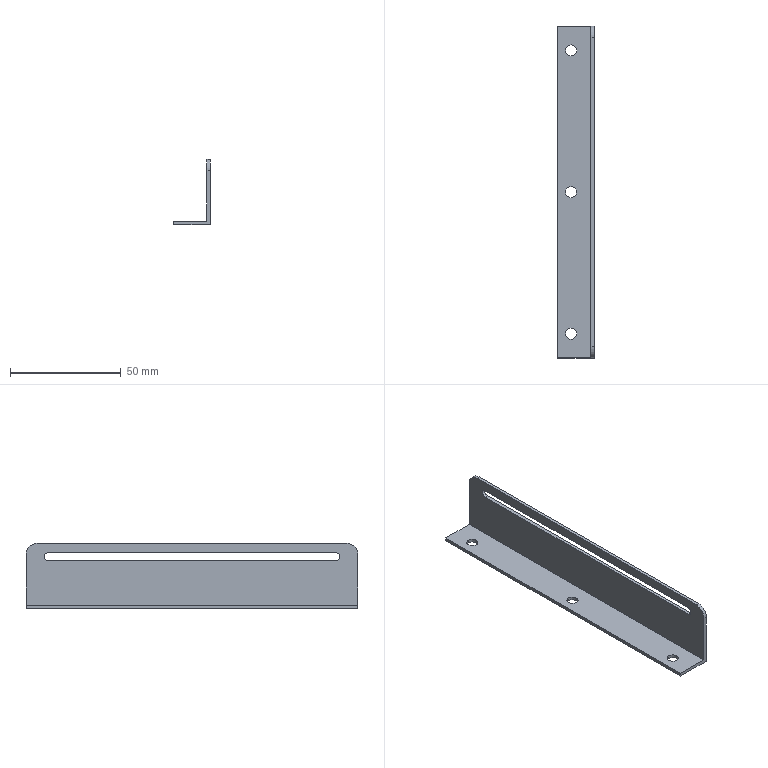Component | SolidWorks | DC-024-31-1 | 1 solid | 20 faces | box 16.5 x 150 x 29.5 mm | volume 9211 mm3 | cylinder 10 | plane 10 | commonest cylinder face diameters 5 x6 3.5 x2 10 x2
build123d program:
from build123d import *

# Parameters (mm, degrees)
EXTRUDE_THIN1_DEPTH      = 75
CUT_EXTRUDE1_DEPTH       = 10
F_5_0_5_DIAMETER_HOLE1_D = 5
FILLET1_R                = 5


with BuildPart() as part:
    # Sketch1 → Extrude-Thin1 (new, symmetric)
    with BuildSketch(Plane.XY):
        Polygon((0, 28), (0, 0), (-15, 0), (-15, -1.5), (1.5, -1.5), (1.5, 28), align=None)
    extrude(amount=EXTRUDE_THIN1_DEPTH, both=True)

    # Sketch2 → Cut-Extrude1 (cut)
    with BuildSketch(Plane.ZY):
        with BuildLine():
            Line((65, 20.25), (-65, 20.25))
            ThreePointArc((-65, 20.25), (-66.75, 22), (-65, 23.75))
            Line((-65, 23.75), (65, 23.75))
            ThreePointArc((65, 23.75), (66.75, 22), (65, 20.25))
        make_face()
    extrude(amount=-CUT_EXTRUDE1_DEPTH, mode=Mode.SUBTRACT)

    # 5.0 _5_ Diameter Hole1 (through all)
    with Locations(Plane(origin=(0, -1.5, 0), x_dir=(-1, 0, 0), z_dir=(0, -1, 0))):
        with Locations((9, 64), (9, 0), (9, -64)):
            Hole(F_5_0_5_DIAMETER_HOLE1_D / 2)

    # Fillet1
    fillet1_edges = [part.edges().sort_by_distance(p)[0] for p in [
        (0.75, 28, 75),
        (0.75, 28, -75),
    ]]
    fillet(fillet1_edges, radius=FILLET1_R)


solid = part.part

# Placed as in the assembly
solid = solid.moved(Location((112.867, 271.909, 14.5), (90, 0, 0)))
STEP:
#1=CARTESIAN_POINT('',(4.089,13.126,0.5709));
#2=VERTEX_POINT('',#1);
#3=CARTESIAN_POINT('',(4.089,13.323,0.5709));
#4=VERTEX_POINT('',#3);
#5=CARTESIAN_POINT('',(4.089,13.225,0.5709));
#6=DIRECTION('',(0.,0.,-1.));
#7=DIRECTION('',(1.,0.,0.));
#8=AXIS2_PLACEMENT_3D('',#5,#6,#7);
#9=CIRCLE('',#8,0.09843);
#10=EDGE_CURVE('',#2,#4,#9,.T.);
#11=ORIENTED_EDGE('',*,*,#10,.F.);
#12=CARTESIAN_POINT('',(4.089,13.126,0.5118));
#13=VERTEX_POINT('',#12);
#14=CARTESIAN_POINT('',(4.089,13.126,0.5118));
#15=DIRECTION('',(0.,0.,-1.));
#16=VECTOR('',#15,39.37);
#17=LINE('',#14,#16);
#18=EDGE_CURVE('',#2,#13,#17,.T.);
#19=ORIENTED_EDGE('',*,*,#18,.T.);
#20=CARTESIAN_POINT('',(4.089,13.323,0.5118));
#21=VERTEX_POINT('',#20);
#22=CARTESIAN_POINT('',(4.089,13.225,0.5118));
#23=DIRECTION('',(0.,0.,-1.));
#24=DIRECTION('',(0.,1.,0.));
#25=AXIS2_PLACEMENT_3D('',#22,#23,#24);
#26=CIRCLE('',#25,0.09843);
#27=EDGE_CURVE('',#13,#21,#26,.T.);
#28=ORIENTED_EDGE('',*,*,#27,.T.);
#29=CARTESIAN_POINT('',(4.089,13.323,0.5118));
#30=DIRECTION('',(0.,0.,-1.));
#31=VECTOR('',#30,39.37);
#32=LINE('',#29,#31);
#33=EDGE_CURVE('',#4,#21,#32,.T.);
#34=ORIENTED_EDGE('',*,*,#33,.F.);
#35=EDGE_LOOP('',(#11,#19,#28,#34));
#36=FACE_OUTER_BOUND('',#35,.T.);
#37=CARTESIAN_POINT('',(4.089,13.225,0.5118));
#38=DIRECTION('',(0.,0.,-1.));
#39=DIRECTION('',(0.,1.,0.));
#40=AXIS2_PLACEMENT_3D('',#37,#38,#39);
#41=CYLINDRICAL_SURFACE('',#40,0.09843);
#42=ADVANCED_FACE('',(#36),#41,.F.);
#43=CARTESIAN_POINT('',(4.089,10.607,0.5709));
#44=VERTEX_POINT('',#43);
#45=CARTESIAN_POINT('',(4.089,10.803,0.5709));
#46=VERTEX_POINT('',#45);
#47=CARTESIAN_POINT('',(4.089,10.705,0.5709));
#48=DIRECTION('',(0.,0.,-1.));
#49=DIRECTION('',(1.,0.,0.));
#50=AXIS2_PLACEMENT_3D('',#47,#48,#49);
#51=CIRCLE('',#50,0.09843);
#52=EDGE_CURVE('',#44,#46,#51,.T.);
#53=ORIENTED_EDGE('',*,*,#52,.F.);
#54=CARTESIAN_POINT('',(4.089,10.607,0.5118));
#55=VERTEX_POINT('',#54);
#56=CARTESIAN_POINT('',(4.089,10.607,0.5118));
#57=DIRECTION('',(0.,0.,-1.));
#58=VECTOR('',#57,39.37);
#59=LINE('',#56,#58);
#60=EDGE_CURVE('',#44,#55,#59,.T.);
#61=ORIENTED_EDGE('',*,*,#60,.T.);
#62=CARTESIAN_POINT('',(4.089,10.803,0.5118));
#63=VERTEX_POINT('',#62);
#64=CARTESIAN_POINT('',(4.089,10.705,0.5118));
#65=DIRECTION('',(0.,0.,-1.));
#66=DIRECTION('',(0.,1.,0.));
#67=AXIS2_PLACEMENT_3D('',#64,#65,#66);
#68=CIRCLE('',#67,0.09843);
#69=EDGE_CURVE('',#55,#63,#68,.T.);
#70=ORIENTED_EDGE('',*,*,#69,.T.);
#71=CARTESIAN_POINT('',(4.089,10.803,0.5118));
#72=DIRECTION('',(0.,0.,-1.));
#73=VECTOR('',#72,39.37);
#74=LINE('',#71,#73);
#75=EDGE_CURVE('',#46,#63,#74,.T.);
#76=ORIENTED_EDGE('',*,*,#75,.F.);
#77=EDGE_LOOP('',(#53,#61,#70,#76));
#78=FACE_OUTER_BOUND('',#77,.T.);
#79=CARTESIAN_POINT('',(4.089,10.705,0.5118));
#80=DIRECTION('',(0.,0.,-1.));
#81=DIRECTION('',(0.,1.,0.));
#82=AXIS2_PLACEMENT_3D('',#79,#80,#81);
#83=CYLINDRICAL_SURFACE('',#82,0.09843);
#84=ADVANCED_FACE('',(#78),#83,.F.);
#85=CARTESIAN_POINT('',(4.089,8.087,0.5709));
#86=VERTEX_POINT('',#85);
#87=CARTESIAN_POINT('',(4.089,8.284,0.5709));
#88=VERTEX_POINT('',#87);
#89=CARTESIAN_POINT('',(4.089,8.185,0.5709));
#90=DIRECTION('',(0.,0.,-1.));
#91=DIRECTION('',(1.,0.,0.));
#92=AXIS2_PLACEMENT_3D('',#89,#90,#91);
#93=CIRCLE('',#92,0.09843);
#94=EDGE_CURVE('',#86,#88,#93,.T.);
#95=ORIENTED_EDGE('',*,*,#94,.F.);
#96=CARTESIAN_POINT('',(4.089,8.087,0.5118));
#97=VERTEX_POINT('',#96);
#98=CARTESIAN_POINT('',(4.089,8.087,0.5118));
#99=DIRECTION('',(0.,0.,-1.));
#100=VECTOR('',#99,39.37);
#101=LINE('',#98,#100);
#102=EDGE_CURVE('',#86,#97,#101,.T.);
#103=ORIENTED_EDGE('',*,*,#102,.T.);
#104=CARTESIAN_POINT('',(4.089,8.284,0.5118));
#105=VERTEX_POINT('',#104);
#106=CARTESIAN_POINT('',(4.089,8.185,0.5118));
#107=DIRECTION('',(0.,0.,-1.));
#108=DIRECTION('',(0.,1.,0.));
#109=AXIS2_PLACEMENT_3D('',#106,#107,#108);
#110=CIRCLE('',#109,0.09843);
#111=EDGE_CURVE('',#97,#105,#110,.T.);
#112=ORIENTED_EDGE('',*,*,#111,.T.);
#113=CARTESIAN_POINT('',(4.089,8.284,0.5118));
#114=DIRECTION('',(0.,0.,-1.));
#115=VECTOR('',#114,39.37);
#116=LINE('',#113,#115);
#117=EDGE_CURVE('',#88,#105,#116,.T.);
#118=ORIENTED_EDGE('',*,*,#117,.F.);
#119=EDGE_LOOP('',(#95,#103,#112,#118));
#120=FACE_OUTER_BOUND('',#119,.T.);
#121=CARTESIAN_POINT('',(4.089,8.185,0.5118));
#122=DIRECTION('',(0.,0.,-1.));
#123=DIRECTION('',(0.,1.,0.));
#124=AXIS2_PLACEMENT_3D('',#121,#122,#123);
#125=CYLINDRICAL_SURFACE('',#124,0.09843);
#126=ADVANCED_FACE('',(#120),#125,.F.);
#127=CARTESIAN_POINT('',(4.089,13.225,0.5709));
#128=DIRECTION('',(0.,0.,-1.));
#129=DIRECTION('',(1.,0.,0.));
#130=AXIS2_PLACEMENT_3D('',#127,#128,#129);
#131=CIRCLE('',#130,0.09843);
#132=EDGE_CURVE('',#4,#2,#131,.T.);
#133=ORIENTED_EDGE('',*,*,#132,.T.);
#134=ORIENTED_EDGE('',*,*,#10,.T.);
#135=EDGE_LOOP('',(#133,#134));
#136=FACE_BOUND('',#135,.T.);
#137=CARTESIAN_POINT('',(4.089,10.705,0.5709));
#138=DIRECTION('',(0.,0.,-1.));
#139=DIRECTION('',(1.,0.,0.));
#140=AXIS2_PLACEMENT_3D('',#137,#138,#139);
#141=CIRCLE('',#140,0.09843);
#142=EDGE_CURVE('',#46,#44,#141,.T.);
#143=ORIENTED_EDGE('',*,*,#142,.T.);
#144=ORIENTED_EDGE('',*,*,#52,.T.);
#145=EDGE_LOOP('',(#143,#144));
#146=FACE_BOUND('',#145,.T.);
#147=CARTESIAN_POINT('',(4.089,8.185,0.5709));
#148=DIRECTION('',(0.,0.,-1.));
#149=DIRECTION('',(1.,0.,0.));
#150=AXIS2_PLACEMENT_3D('',#147,#148,#149);
#151=CIRCLE('',#150,0.09843);
#152=EDGE_CURVE('',#88,#86,#151,.T.);
#153=ORIENTED_EDGE('',*,*,#152,.T.);
#154=ORIENTED_EDGE('',*,*,#94,.T.);
#155=EDGE_LOOP('',(#153,#154));
#156=FACE_BOUND('',#155,.T.);
#157=CARTESIAN_POINT('',(4.444,13.658,0.5709));
#158=VERTEX_POINT('',#157);
#159=CARTESIAN_POINT('',(3.853,13.658,0.5709));
#160=VERTEX_POINT('',#159);
#161=CARTESIAN_POINT('',(4.444,13.658,0.5709));
#162=DIRECTION('',(-1.,0.,-0.));
#163=VECTOR('',#162,39.37);
#164=LINE('',#161,#163);
#165=EDGE_CURVE('',#158,#160,#164,.T.);
#166=ORIENTED_EDGE('',*,*,#165,.T.);
#167=CARTESIAN_POINT('',(3.853,7.752,0.5709));
#168=VERTEX_POINT('',#167);
#169=CARTESIAN_POINT('',(3.853,7.752,0.5709));
#170=DIRECTION('',(0.,1.,0.));
#171=VECTOR('',#170,39.37);
#172=LINE('',#169,#171);
#173=EDGE_CURVE('',#168,#160,#172,.T.);
#174=ORIENTED_EDGE('',*,*,#173,.F.);
#175=CARTESIAN_POINT('',(4.444,7.752,0.5709));
#176=VERTEX_POINT('',#175);
#177=CARTESIAN_POINT('',(4.444,7.752,0.5709));
#178=DIRECTION('',(-1.,0.,-0.));
#179=VECTOR('',#178,39.37);
#180=LINE('',#177,#179);
#181=EDGE_CURVE('',#176,#168,#180,.T.);
#182=ORIENTED_EDGE('',*,*,#181,.F.);
#183=CARTESIAN_POINT('',(4.444,7.752,0.5709));
#184=DIRECTION('',(0.,1.,0.));
#185=VECTOR('',#184,39.37);
#186=LINE('',#183,#185);
#187=EDGE_CURVE('',#176,#158,#186,.T.);
#188=ORIENTED_EDGE('',*,*,#187,.T.);
#189=EDGE_LOOP('',(#166,#174,#182,#188));
#190=FACE_OUTER_BOUND('',#189,.T.);
#191=CARTESIAN_POINT('',(4.444,7.752,0.5709));
#192=DIRECTION('',(0.,0.,-1.));
#193=DIRECTION('',(1.,0.,0.));
#194=AXIS2_PLACEMENT_3D('',#191,#192,#193);
#195=PLANE('',#194);
#196=ADVANCED_FACE('',(#136,#146,#156,#190),#195,.F.);
#197=CARTESIAN_POINT('',(3.853,13.658,0.5118));
#198=VERTEX_POINT('',#197);
#199=CARTESIAN_POINT('',(3.853,13.658,0.5118));
#200=DIRECTION('',(0.,0.,1.));
#201=VECTOR('',#200,39.37);
#202=LINE('',#199,#201);
#203=EDGE_CURVE('',#198,#160,#202,.T.);
#204=ORIENTED_EDGE('',*,*,#203,.F.);
#205=CARTESIAN_POINT('',(3.853,7.752,0.5118));
#206=VERTEX_POINT('',#205);
#207=CARTESIAN_POINT('',(3.853,7.752,0.5118));
#208=DIRECTION('',(0.,1.,0.));
#209=VECTOR('',#208,39.37);
#210=LINE('',#207,#209);
#211=EDGE_CURVE('',#206,#198,#210,.T.);
#212=ORIENTED_EDGE('',*,*,#211,.F.);
#213=CARTESIAN_POINT('',(3.853,7.752,0.5118));
#214=DIRECTION('',(0.,0.,1.));
#215=VECTOR('',#214,39.37);
#216=LINE('',#213,#215);
#217=EDGE_CURVE('',#206,#168,#216,.T.);
#218=ORIENTED_EDGE('',*,*,#217,.T.);
#219=ORIENTED_EDGE('',*,*,#173,.T.);
#220=EDGE_LOOP('',(#204,#212,#218,#219));
#221=FACE_OUTER_BOUND('',#220,.T.);
#222=CARTESIAN_POINT('',(3.853,7.752,0.5118));
#223=DIRECTION('',(-1.,0.,0.));
#224=DIRECTION('',(0.,-1.,0.));
#225=AXIS2_PLACEMENT_3D('',#222,#223,#224);
#226=PLANE('',#225);
#227=ADVANCED_FACE('',(#221),#226,.T.);
#228=CARTESIAN_POINT('',(4.089,13.225,0.5118));
#229=DIRECTION('',(0.,0.,-1.));
#230=DIRECTION('',(0.,1.,0.));
#231=AXIS2_PLACEMENT_3D('',#228,#229,#230);
#232=CIRCLE('',#231,0.09843);
#233=EDGE_CURVE('',#21,#13,#232,.T.);
#234=ORIENTED_EDGE('',*,*,#233,.F.);
#235=ORIENTED_EDGE('',*,*,#27,.F.);
#236=EDGE_LOOP('',(#234,#235));
#237=FACE_BOUND('',#236,.T.);
#238=CARTESIAN_POINT('',(4.089,10.705,0.5118));
#239=DIRECTION('',(0.,0.,-1.));
#240=DIRECTION('',(0.,1.,0.));
#241=AXIS2_PLACEMENT_3D('',#238,#239,#240);
#242=CIRCLE('',#241,0.09843);
#243=EDGE_CURVE('',#63,#55,#242,.T.);
#244=ORIENTED_EDGE('',*,*,#243,.F.);
#245=ORIENTED_EDGE('',*,*,#69,.F.);
#246=EDGE_LOOP('',(#244,#245));
#247=FACE_BOUND('',#246,.T.);
#248=CARTESIAN_POINT('',(4.089,8.185,0.5118));
#249=DIRECTION('',(0.,0.,-1.));
#250=DIRECTION('',(0.,1.,0.));
#251=AXIS2_PLACEMENT_3D('',#248,#249,#250);
#252=CIRCLE('',#251,0.09843);
#253=EDGE_CURVE('',#105,#97,#252,.T.);
#254=ORIENTED_EDGE('',*,*,#253,.F.);
#255=ORIENTED_EDGE('',*,*,#111,.F.);
#256=EDGE_LOOP('',(#254,#255));
#257=FACE_BOUND('',#256,.T.);
#258=CARTESIAN_POINT('',(4.503,13.658,0.5118));
#259=VERTEX_POINT('',#258);
#260=CARTESIAN_POINT('',(4.444,13.658,0.5118));
#261=DIRECTION('',(-1.,0.,-0.));
#262=VECTOR('',#261,39.37);
#263=LINE('',#260,#262);
#264=EDGE_CURVE('',#259,#198,#263,.T.);
#265=ORIENTED_EDGE('',*,*,#264,.F.);
#266=CARTESIAN_POINT('',(4.503,7.752,0.5118));
#267=VERTEX_POINT('',#266);
#268=CARTESIAN_POINT('',(4.503,7.752,0.5118));
#269=DIRECTION('',(0.,1.,0.));
#270=VECTOR('',#269,39.37);
#271=LINE('',#268,#270);
#272=EDGE_CURVE('',#267,#259,#271,.T.);
#273=ORIENTED_EDGE('',*,*,#272,.F.);
#274=CARTESIAN_POINT('',(4.444,7.752,0.5118));
#275=DIRECTION('',(-1.,0.,-0.));
#276=VECTOR('',#275,39.37);
#277=LINE('',#274,#276);
#278=EDGE_CURVE('',#267,#206,#277,.T.);
#279=ORIENTED_EDGE('',*,*,#278,.T.);
#280=ORIENTED_EDGE('',*,*,#211,.T.);
#281=EDGE_LOOP('',(#265,#273,#279,#280));
#282=FACE_OUTER_BOUND('',#281,.T.);
#283=CARTESIAN_POINT('',(4.444,7.752,0.5118));
#284=DIRECTION('',(0.,0.,-1.));
#285=DIRECTION('',(1.,0.,0.));
#286=AXIS2_PLACEMENT_3D('',#283,#284,#285);
#287=PLANE('',#286);
#288=ADVANCED_FACE('',(#237,#247,#257,#282),#287,.T.);
#289=CARTESIAN_POINT('',(4.503,8.146,1.506));
#290=VERTEX_POINT('',#289);
#291=CARTESIAN_POINT('',(4.503,8.146,1.368));
#292=VERTEX_POINT('',#291);
#293=CARTESIAN_POINT('',(4.503,8.146,1.437));
#294=DIRECTION('',(1.,0.,0.));
#295=DIRECTION('',(0.,0.,1.));
#296=AXIS2_PLACEMENT_3D('',#293,#294,#295);
#297=CIRCLE('',#296,0.0689);
#298=EDGE_CURVE('',#290,#292,#297,.T.);
#299=ORIENTED_EDGE('',*,*,#298,.F.);
#300=CARTESIAN_POINT('',(4.503,13.264,1.506));
#301=VERTEX_POINT('',#300);
#302=CARTESIAN_POINT('',(4.503,7.752,1.506));
#303=DIRECTION('',(0.,-1.,0.));
#304=VECTOR('',#303,39.37);
#305=LINE('',#302,#304);
#306=EDGE_CURVE('',#301,#290,#305,.T.);
#307=ORIENTED_EDGE('',*,*,#306,.F.);
#308=CARTESIAN_POINT('',(4.503,13.264,1.368));
#309=VERTEX_POINT('',#308);
#310=CARTESIAN_POINT('',(4.503,13.264,1.437));
#311=DIRECTION('',(1.,0.,0.));
#312=DIRECTION('',(0.,0.,1.));
#313=AXIS2_PLACEMENT_3D('',#310,#311,#312);
#314=CIRCLE('',#313,0.0689);
#315=EDGE_CURVE('',#309,#301,#314,.T.);
#316=ORIENTED_EDGE('',*,*,#315,.F.);
#317=CARTESIAN_POINT('',(4.503,7.752,1.368));
#318=DIRECTION('',(0.,1.,-0.));
#319=VECTOR('',#318,39.37);
#320=LINE('',#317,#319);
#321=EDGE_CURVE('',#292,#309,#320,.T.);
#322=ORIENTED_EDGE('',*,*,#321,.F.);
#323=EDGE_LOOP('',(#299,#307,#316,#322));
#324=FACE_BOUND('',#323,.T.);
#325=CARTESIAN_POINT('',(4.503,13.658,1.476));
#326=VERTEX_POINT('',#325);
#327=CARTESIAN_POINT('',(4.503,13.658,1.673));
#328=DIRECTION('',(0.,0.,-1.));
#329=VECTOR('',#328,39.37);
#330=LINE('',#327,#329);
#331=EDGE_CURVE('',#326,#259,#330,.T.);
#332=ORIENTED_EDGE('',*,*,#331,.F.);
#333=CARTESIAN_POINT('',(4.503,13.461,1.673));
#334=VERTEX_POINT('',#333);
#335=CARTESIAN_POINT('',(4.503,13.461,1.476));
#336=DIRECTION('',(1.,0.,0.));
#337=DIRECTION('',(0.,0.,1.));
#338=AXIS2_PLACEMENT_3D('',#335,#336,#337);
#339=CIRCLE('',#338,0.1969);
#340=EDGE_CURVE('',#326,#334,#339,.T.);
#341=ORIENTED_EDGE('',*,*,#340,.T.);
#342=CARTESIAN_POINT('',(4.503,7.949,1.673));
#343=VERTEX_POINT('',#342);
#344=CARTESIAN_POINT('',(4.503,7.752,1.673));
#345=DIRECTION('',(0.,1.,0.));
#346=VECTOR('',#345,39.37);
#347=LINE('',#344,#346);
#348=EDGE_CURVE('',#343,#334,#347,.T.);
#349=ORIENTED_EDGE('',*,*,#348,.F.);
#350=CARTESIAN_POINT('',(4.503,7.752,1.476));
#351=VERTEX_POINT('',#350);
#352=CARTESIAN_POINT('',(4.503,7.949,1.476));
#353=DIRECTION('',(1.,0.,0.));
#354=DIRECTION('',(0.,0.,1.));
#355=AXIS2_PLACEMENT_3D('',#352,#353,#354);
#356=CIRCLE('',#355,0.1969);
#357=EDGE_CURVE('',#343,#351,#356,.T.);
#358=ORIENTED_EDGE('',*,*,#357,.T.);
#359=CARTESIAN_POINT('',(4.503,7.752,1.673));
#360=DIRECTION('',(0.,0.,-1.));
#361=VECTOR('',#360,39.37);
#362=LINE('',#359,#361);
#363=EDGE_CURVE('',#351,#267,#362,.T.);
#364=ORIENTED_EDGE('',*,*,#363,.T.);
#365=ORIENTED_EDGE('',*,*,#272,.T.);
#366=EDGE_LOOP('',(#332,#341,#349,#358,#364,#365));
#367=FACE_OUTER_BOUND('',#366,.T.);
#368=CARTESIAN_POINT('',(4.503,7.752,1.673));
#369=DIRECTION('',(1.,0.,0.));
#370=DIRECTION('',(-0.,0.,1.));
#371=AXIS2_PLACEMENT_3D('',#368,#369,#370);
#372=PLANE('',#371);
#373=ADVANCED_FACE('',(#324,#367),#372,.T.);
#374=ORIENTED_EDGE('',*,*,#348,.T.);
#375=CARTESIAN_POINT('',(4.444,13.461,1.673));
#376=VERTEX_POINT('',#375);
#377=CARTESIAN_POINT('',(4.444,13.461,1.673));
#378=DIRECTION('',(-1.,0.,0.));
#379=VECTOR('',#378,39.37);
#380=LINE('',#377,#379);
#381=EDGE_CURVE('',#334,#376,#380,.T.);
#382=ORIENTED_EDGE('',*,*,#381,.T.);
#383=CARTESIAN_POINT('',(4.444,7.949,1.673));
#384=VERTEX_POINT('',#383);
#385=CARTESIAN_POINT('',(4.444,7.752,1.673));
#386=DIRECTION('',(0.,1.,0.));
#387=VECTOR('',#386,39.37);
#388=LINE('',#385,#387);
#389=EDGE_CURVE('',#384,#376,#388,.T.);
#390=ORIENTED_EDGE('',*,*,#389,.F.);
#391=CARTESIAN_POINT('',(4.503,7.949,1.673));
#392=DIRECTION('',(1.,0.,0.));
#393=VECTOR('',#392,39.37);
#394=LINE('',#391,#393);
#395=EDGE_CURVE('',#384,#343,#394,.T.);
#396=ORIENTED_EDGE('',*,*,#395,.T.);
#397=EDGE_LOOP('',(#374,#382,#390,#396));
#398=FACE_OUTER_BOUND('',#397,.T.);
#399=CARTESIAN_POINT('',(4.444,7.752,1.673));
#400=DIRECTION('',(0.,0.,1.));
#401=DIRECTION('',(0.,-1.,0.));
#402=AXIS2_PLACEMENT_3D('',#399,#400,#401);
#403=PLANE('',#402);
#404=ADVANCED_FACE('',(#398),#403,.T.);
#405=CARTESIAN_POINT('',(4.444,8.146,1.506));
#406=VERTEX_POINT('',#405);
#407=CARTESIAN_POINT('',(4.444,13.264,1.506));
#408=VERTEX_POINT('',#407);
#409=CARTESIAN_POINT('',(4.444,8.146,1.506));
#410=DIRECTION('',(0.,1.,0.));
#411=VECTOR('',#410,39.37);
#412=LINE('',#409,#411);
#413=EDGE_CURVE('',#406,#408,#412,.T.);
#414=ORIENTED_EDGE('',*,*,#413,.F.);
#415=CARTESIAN_POINT('',(4.444,8.146,1.368));
#416=VERTEX_POINT('',#415);
#417=CARTESIAN_POINT('',(4.444,8.146,1.437));
#418=DIRECTION('',(-1.,0.,0.));
#419=DIRECTION('',(0.,0.,-1.));
#420=AXIS2_PLACEMENT_3D('',#417,#418,#419);
#421=CIRCLE('',#420,0.0689);
#422=EDGE_CURVE('',#416,#406,#421,.T.);
#423=ORIENTED_EDGE('',*,*,#422,.F.);
#424=CARTESIAN_POINT('',(4.444,13.264,1.368));
#425=VERTEX_POINT('',#424);
#426=CARTESIAN_POINT('',(4.444,8.146,1.368));
#427=DIRECTION('',(0.,-1.,0.));
#428=VECTOR('',#427,39.37);
#429=LINE('',#426,#428);
#430=EDGE_CURVE('',#425,#416,#429,.T.);
#431=ORIENTED_EDGE('',*,*,#430,.F.);
#432=CARTESIAN_POINT('',(4.444,13.264,1.437));
#433=DIRECTION('',(-1.,0.,0.));
#434=DIRECTION('',(0.,0.,-1.));
#435=AXIS2_PLACEMENT_3D('',#432,#433,#434);
#436=CIRCLE('',#435,0.0689);
#437=EDGE_CURVE('',#408,#425,#436,.T.);
#438=ORIENTED_EDGE('',*,*,#437,.F.);
#439=EDGE_LOOP('',(#414,#423,#431,#438));
#440=FACE_BOUND('',#439,.T.);
#441=ORIENTED_EDGE('',*,*,#389,.T.);
#442=CARTESIAN_POINT('',(4.444,13.658,1.476));
#443=VERTEX_POINT('',#442);
#444=CARTESIAN_POINT('',(4.444,13.461,1.476));
#445=DIRECTION('',(-1.,0.,-0.));
#446=DIRECTION('',(0.,0.,1.));
#447=AXIS2_PLACEMENT_3D('',#444,#445,#446);
#448=CIRCLE('',#447,0.1969);
#449=EDGE_CURVE('',#376,#443,#448,.T.);
#450=ORIENTED_EDGE('',*,*,#449,.T.);
#451=CARTESIAN_POINT('',(4.444,13.658,1.673));
#452=DIRECTION('',(0.,0.,-1.));
#453=VECTOR('',#452,39.37);
#454=LINE('',#451,#453);
#455=EDGE_CURVE('',#443,#158,#454,.T.);
#456=ORIENTED_EDGE('',*,*,#455,.T.);
#457=ORIENTED_EDGE('',*,*,#187,.F.);
#458=CARTESIAN_POINT('',(4.444,7.752,1.476));
#459=VERTEX_POINT('',#458);
#460=CARTESIAN_POINT('',(4.444,7.752,1.673));
#461=DIRECTION('',(0.,0.,-1.));
#462=VECTOR('',#461,39.37);
#463=LINE('',#460,#462);
#464=EDGE_CURVE('',#459,#176,#463,.T.);
#465=ORIENTED_EDGE('',*,*,#464,.F.);
#466=CARTESIAN_POINT('',(4.444,7.949,1.476));
#467=DIRECTION('',(-1.,0.,-0.));
#468=DIRECTION('',(0.,0.,1.));
#469=AXIS2_PLACEMENT_3D('',#466,#467,#468);
#470=CIRCLE('',#469,0.1969);
#471=EDGE_CURVE('',#459,#384,#470,.T.);
#472=ORIENTED_EDGE('',*,*,#471,.T.);
#473=EDGE_LOOP('',(#441,#450,#456,#457,#465,#472));
#474=FACE_OUTER_BOUND('',#473,.T.);
#475=CARTESIAN_POINT('',(4.444,7.752,1.673));
#476=DIRECTION('',(1.,0.,0.));
#477=DIRECTION('',(-0.,0.,1.));
#478=AXIS2_PLACEMENT_3D('',#475,#476,#477);
#479=PLANE('',#478);
#480=ADVANCED_FACE('',(#440,#474),#479,.F.);
#481=ORIENTED_EDGE('',*,*,#363,.F.);
#482=CARTESIAN_POINT('',(4.444,7.752,1.476));
#483=DIRECTION('',(-1.,0.,0.));
#484=VECTOR('',#483,39.37);
#485=LINE('',#482,#484);
#486=EDGE_CURVE('',#351,#459,#485,.T.);
#487=ORIENTED_EDGE('',*,*,#486,.T.);
#488=ORIENTED_EDGE('',*,*,#464,.T.);
#489=ORIENTED_EDGE('',*,*,#181,.T.);
#490=ORIENTED_EDGE('',*,*,#217,.F.);
#491=ORIENTED_EDGE('',*,*,#278,.F.);
#492=EDGE_LOOP('',(#481,#487,#488,#489,#490,#491));
#493=FACE_OUTER_BOUND('',#492,.T.);
#494=CARTESIAN_POINT('',(4.444,7.752,0.5709));
#495=DIRECTION('',(0.,1.,0.));
#496=DIRECTION('',(-1.,0.,0.));
#497=AXIS2_PLACEMENT_3D('',#494,#495,#496);
#498=PLANE('',#497);
#499=ADVANCED_FACE('',(#493),#498,.F.);
#500=ORIENTED_EDGE('',*,*,#455,.F.);
#501=CARTESIAN_POINT('',(4.444,13.658,1.476));
#502=DIRECTION('',(1.,0.,0.));
#503=VECTOR('',#502,39.37);
#504=LINE('',#501,#503);
#505=EDGE_CURVE('',#443,#326,#504,.T.);
#506=ORIENTED_EDGE('',*,*,#505,.T.);
#507=ORIENTED_EDGE('',*,*,#331,.T.);
#508=ORIENTED_EDGE('',*,*,#264,.T.);
#509=ORIENTED_EDGE('',*,*,#203,.T.);
#510=ORIENTED_EDGE('',*,*,#165,.F.);
#511=EDGE_LOOP('',(#500,#506,#507,#508,#509,#510));
#512=FACE_OUTER_BOUND('',#511,.T.);
#513=CARTESIAN_POINT('',(4.444,13.658,0.5709));
#514=DIRECTION('',(0.,1.,0.));
#515=DIRECTION('',(-1.,0.,0.));
#516=AXIS2_PLACEMENT_3D('',#513,#514,#515);
#517=PLANE('',#516);
#518=ADVANCED_FACE('',(#512),#517,.T.);
#519=ORIENTED_EDGE('',*,*,#298,.T.);
#520=CARTESIAN_POINT('',(4.837,8.146,1.368));
#521=DIRECTION('',(-1.,0.,0.));
#522=VECTOR('',#521,39.37);
#523=LINE('',#520,#522);
#524=EDGE_CURVE('',#292,#416,#523,.T.);
#525=ORIENTED_EDGE('',*,*,#524,.T.);
#526=ORIENTED_EDGE('',*,*,#422,.T.);
#527=CARTESIAN_POINT('',(4.837,8.146,1.506));
#528=DIRECTION('',(-1.,0.,0.));
#529=VECTOR('',#528,39.37);
#530=LINE('',#527,#529);
#531=EDGE_CURVE('',#290,#406,#530,.T.);
#532=ORIENTED_EDGE('',*,*,#531,.F.);
#533=EDGE_LOOP('',(#519,#525,#526,#532));
#534=FACE_OUTER_BOUND('',#533,.T.);
#535=CARTESIAN_POINT('',(4.837,8.146,1.437));
#536=DIRECTION('',(-1.,0.,0.));
#537=DIRECTION('',(0.,0.,-1.));
#538=AXIS2_PLACEMENT_3D('',#535,#536,#537);
#539=CYLINDRICAL_SURFACE('',#538,0.0689);
#540=ADVANCED_FACE('',(#534),#539,.F.);
#541=ORIENTED_EDGE('',*,*,#321,.T.);
#542=CARTESIAN_POINT('',(4.837,13.264,1.368));
#543=DIRECTION('',(-1.,0.,0.));
#544=VECTOR('',#543,39.37);
#545=LINE('',#542,#544);
#546=EDGE_CURVE('',#309,#425,#545,.T.);
#547=ORIENTED_EDGE('',*,*,#546,.T.);
#548=ORIENTED_EDGE('',*,*,#430,.T.);
#549=ORIENTED_EDGE('',*,*,#524,.F.);
#550=EDGE_LOOP('',(#541,#547,#548,#549));
#551=FACE_OUTER_BOUND('',#550,.T.);
#552=CARTESIAN_POINT('',(4.837,8.146,1.368));
#553=DIRECTION('',(-0.,-0.,-1.));
#554=DIRECTION('',(0.,1.,-0.));
#555=AXIS2_PLACEMENT_3D('',#552,#553,#554);
#556=PLANE('',#555);
#557=ADVANCED_FACE('',(#551),#556,.F.);
#558=ORIENTED_EDGE('',*,*,#315,.T.);
#559=CARTESIAN_POINT('',(4.837,13.264,1.506));
#560=DIRECTION('',(-1.,0.,0.));
#561=VECTOR('',#560,39.37);
#562=LINE('',#559,#561);
#563=EDGE_CURVE('',#301,#408,#562,.T.);
#564=ORIENTED_EDGE('',*,*,#563,.T.);
#565=ORIENTED_EDGE('',*,*,#437,.T.);
#566=ORIENTED_EDGE('',*,*,#546,.F.);
#567=EDGE_LOOP('',(#558,#564,#565,#566));
#568=FACE_OUTER_BOUND('',#567,.T.);
#569=CARTESIAN_POINT('',(4.837,13.264,1.437));
#570=DIRECTION('',(-1.,0.,0.));
#571=DIRECTION('',(0.,0.,-1.));
#572=AXIS2_PLACEMENT_3D('',#569,#570,#571);
#573=CYLINDRICAL_SURFACE('',#572,0.0689);
#574=ADVANCED_FACE('',(#568),#573,.F.);
#575=ORIENTED_EDGE('',*,*,#306,.T.);
#576=ORIENTED_EDGE('',*,*,#531,.T.);
#577=ORIENTED_EDGE('',*,*,#413,.T.);
#578=ORIENTED_EDGE('',*,*,#563,.F.);
#579=EDGE_LOOP('',(#575,#576,#577,#578));
#580=FACE_OUTER_BOUND('',#579,.T.);
#581=CARTESIAN_POINT('',(4.837,8.146,1.506));
#582=DIRECTION('',(0.,0.,1.));
#583=DIRECTION('',(-1.,0.,0.));
#584=AXIS2_PLACEMENT_3D('',#581,#582,#583);
#585=PLANE('',#584);
#586=ADVANCED_FACE('',(#580),#585,.F.);
#587=ORIENTED_EDGE('',*,*,#102,.F.);
#588=ORIENTED_EDGE('',*,*,#152,.F.);
#589=ORIENTED_EDGE('',*,*,#117,.T.);
#590=ORIENTED_EDGE('',*,*,#253,.T.);
#591=EDGE_LOOP('',(#587,#588,#589,#590));
#592=FACE_OUTER_BOUND('',#591,.T.);
#593=CARTESIAN_POINT('',(4.089,8.185,0.5118));
#594=DIRECTION('',(0.,0.,-1.));
#595=DIRECTION('',(0.,1.,0.));
#596=AXIS2_PLACEMENT_3D('',#593,#594,#595);
#597=CYLINDRICAL_SURFACE('',#596,0.09843);
#598=ADVANCED_FACE('',(#592),#597,.F.);
#599=ORIENTED_EDGE('',*,*,#60,.F.);
#600=ORIENTED_EDGE('',*,*,#142,.F.);
#601=ORIENTED_EDGE('',*,*,#75,.T.);
#602=ORIENTED_EDGE('',*,*,#243,.T.);
#603=EDGE_LOOP('',(#599,#600,#601,#602));
#604=FACE_OUTER_BOUND('',#603,.T.);
#605=CARTESIAN_POINT('',(4.089,10.705,0.5118));
#606=DIRECTION('',(0.,0.,-1.));
#607=DIRECTION('',(0.,1.,0.));
#608=AXIS2_PLACEMENT_3D('',#605,#606,#607);
#609=CYLINDRICAL_SURFACE('',#608,0.09843);
#610=ADVANCED_FACE('',(#604),#609,.F.);
#611=ORIENTED_EDGE('',*,*,#18,.F.);
#612=ORIENTED_EDGE('',*,*,#132,.F.);
#613=ORIENTED_EDGE('',*,*,#33,.T.);
#614=ORIENTED_EDGE('',*,*,#233,.T.);
#615=EDGE_LOOP('',(#611,#612,#613,#614));
#616=FACE_OUTER_BOUND('',#615,.T.);
#617=CARTESIAN_POINT('',(4.089,13.225,0.5118));
#618=DIRECTION('',(0.,0.,-1.));
#619=DIRECTION('',(0.,1.,0.));
#620=AXIS2_PLACEMENT_3D('',#617,#618,#619);
#621=CYLINDRICAL_SURFACE('',#620,0.09843);
#622=ADVANCED_FACE('',(#616),#621,.F.);
#623=ORIENTED_EDGE('',*,*,#449,.F.);
#624=ORIENTED_EDGE('',*,*,#381,.F.);
#625=ORIENTED_EDGE('',*,*,#340,.F.);
#626=ORIENTED_EDGE('',*,*,#505,.F.);
#627=EDGE_LOOP('',(#623,#624,#625,#626));
#628=FACE_OUTER_BOUND('',#627,.T.);
#629=CARTESIAN_POINT('',(4.444,13.461,1.476));
#630=DIRECTION('',(1.,0.,0.));
#631=DIRECTION('',(0.,1.,0.));
#632=AXIS2_PLACEMENT_3D('',#629,#630,#631);
#633=CYLINDRICAL_SURFACE('',#632,0.1969);
#634=ADVANCED_FACE('',(#628),#633,.T.);
#635=ORIENTED_EDGE('',*,*,#471,.F.);
#636=ORIENTED_EDGE('',*,*,#486,.F.);
#637=ORIENTED_EDGE('',*,*,#357,.F.);
#638=ORIENTED_EDGE('',*,*,#395,.F.);
#639=EDGE_LOOP('',(#635,#636,#637,#638));
#640=FACE_OUTER_BOUND('',#639,.T.);
#641=CARTESIAN_POINT('',(4.444,7.949,1.476));
#642=DIRECTION('',(-1.,0.,0.));
#643=DIRECTION('',(0.,-1.,0.));
#644=AXIS2_PLACEMENT_3D('',#641,#642,#643);
#645=CYLINDRICAL_SURFACE('',#644,0.1969);
#646=ADVANCED_FACE('',(#640),#645,.T.);
#647=CLOSED_SHELL('',(#42,#84,#126,#196,#227,#288,#373,#404,#480,#499,#518,#540,#557,#574,#586,#598,#610,#622,#634,#646));
#648=MANIFOLD_SOLID_BREP('',#647);
#649=CARTESIAN_POINT('',(0.,0.,0.));
#650=DIRECTION('',(0.,0.,1.));
#651=DIRECTION('',(1.,0.,0.));
#652=AXIS2_PLACEMENT_3D('',#649,#650,#651);
#653=(LENGTH_UNIT()NAMED_UNIT(*)SI_UNIT($,.METRE.));
#654=LENGTH_MEASURE_WITH_UNIT(LENGTH_MEASURE(0.0254),#653);
#655=DIMENSIONAL_EXPONENTS(1.,0.,0.,0.,0.,0.,0.);
#656=(CONVERSION_BASED_UNIT('',#654)LENGTH_UNIT()NAMED_UNIT(#655));
#657=UNCERTAINTY_MEASURE_WITH_UNIT(LENGTH_MEASURE(0.00001),#656,'','');
#658=(NAMED_UNIT(*)PLANE_ANGLE_UNIT()SI_UNIT($,.RADIAN.));
#659=(NAMED_UNIT(*)SI_UNIT($,.STERADIAN.)SOLID_ANGLE_UNIT());
#660=(GEOMETRIC_REPRESENTATION_CONTEXT(3)GLOBAL_UNCERTAINTY_ASSIGNED_CONTEXT((#657))GLOBAL_UNIT_ASSIGNED_CONTEXT((#656,#658,#659))REPRESENTATION_CONTEXT('',''));
#661=ADVANCED_BREP_SHAPE_REPRESENTATION('',(#648,#652),#660);
#662=COLOUR_RGB('',0.7922,0.8196,0.9333);
#663=FILL_AREA_STYLE_COLOUR('',#662);
#664=FILL_AREA_STYLE('',(#663));
#665=SURFACE_STYLE_FILL_AREA(#664);
#666=SURFACE_SIDE_STYLE('',(#665));
#667=SURFACE_STYLE_USAGE(.BOTH.,#666);
#668=PRESENTATION_STYLE_ASSIGNMENT((#667));
#669=STYLED_ITEM('',(#668),#648);
#670=PRESENTATION_LAYER_ASSIGNMENT('','',(#669));
#671=(LENGTH_UNIT()NAMED_UNIT(*)SI_UNIT($,.METRE.));
#672=LENGTH_MEASURE_WITH_UNIT(LENGTH_MEASURE(0.0254),#671);
#673=DIMENSIONAL_EXPONENTS(1.,0.,0.,0.,0.,0.,0.);
#674=(CONVERSION_BASED_UNIT('',#672)LENGTH_UNIT()NAMED_UNIT(#673));
#675=UNCERTAINTY_MEASURE_WITH_UNIT(LENGTH_MEASURE(0.00001),#674,'','');
#676=(NAMED_UNIT(*)PLANE_ANGLE_UNIT()SI_UNIT($,.RADIAN.));
#677=(NAMED_UNIT(*)SI_UNIT($,.STERADIAN.)SOLID_ANGLE_UNIT());
#678=(GEOMETRIC_REPRESENTATION_CONTEXT(3)GLOBAL_UNCERTAINTY_ASSIGNED_CONTEXT((#675))GLOBAL_UNIT_ASSIGNED_CONTEXT((#674,#676,#677))REPRESENTATION_CONTEXT('',''));
#679=MECHANICAL_DESIGN_GEOMETRIC_PRESENTATION_REPRESENTATION('',(#669),#678);